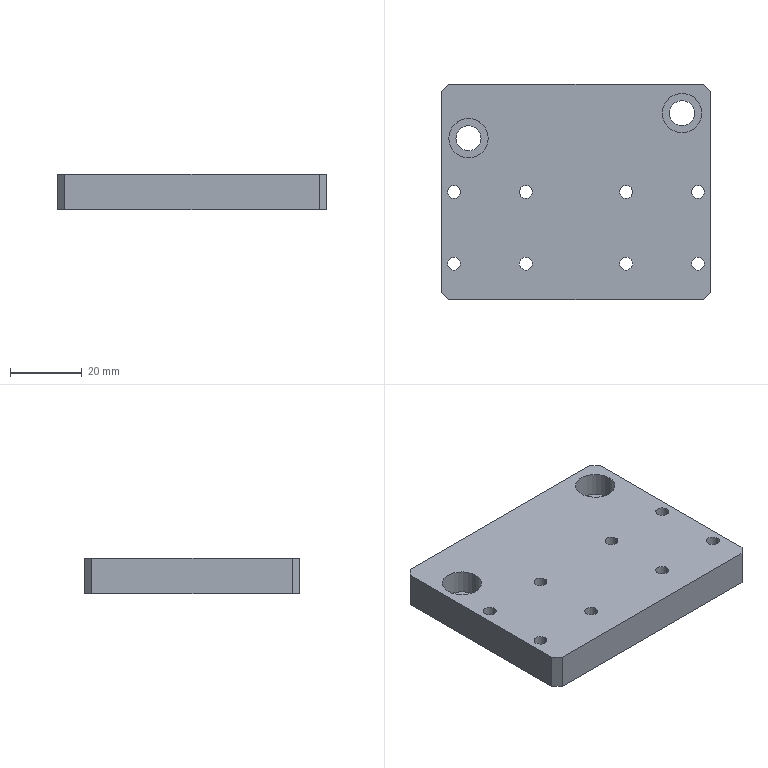Component | SolidWorks | 8TC-A17001-90-03PressureRollerMountingPlate2-1 | 1 solid | 64 faces | box 75 x 60 x 10 mm | volume 41711 mm3 | cylinder 42 | plane 20 | cone 2 | commonest cylinder face diameters 6 x16 3.6 x16 11 x4 7 x4 5 x2 | material A3
build123d program:
from build123d import *

# Parameters (mm, degrees)
SKETCH1_W                                         = 75
SKETCH1_H                                         = 60
BOSS_EXTRUDE1_DEPTH                               = 10
HOLE_SIZE_ACCORDING_TO_HEXAGON_SOCKET_D           = 3.6
HOLE_SIZE_ACCORDING_TO_HEXAGON_SOCKET_CBORE_D     = 6
HOLE_SIZE_ACCORDING_TO_HEXAGON_SOCKET_CBORE_DEPTH = 3.4
HOLE_SIZE_ACCORDING_TO_HEXAGON_SO_2_D             = 7
HOLE_SIZE_ACCORDING_TO_HEXAGON_SO_2_CBORE_D       = 11
HOLE_SIZE_ACCORDING_TO_HEXAGON_SO_2_CBORE_DEPTH   = 6.8
CHAMFER1_SIZE                                     = 2
M6_TAPPED_HOLE1_D                                 = 5
M6_TAPPED_HOLE1_DEPTH                             = 18
M6_TAPPED_HOLE1_TIP                               = 1.502


with BuildPart() as part:
    # Sketch1 → Boss-Extrude1 (new body)
    with BuildSketch(Plane.XY):
        Rectangle(SKETCH1_W, SKETCH1_H)
    extrude(amount=BOSS_EXTRUDE1_DEPTH)

    # Hole Size _ according to_ Hexagon Socket (through all)
    with Locations(Plane.XY.offset(10)):
        with Locations((-34, 20), (-34, 0), (-14, 20), (-14, 0), (14, 20), (34, 20), (14, 0), (34, 0)):
            CounterBoreHole(HOLE_SIZE_ACCORDING_TO_HEXAGON_SOCKET_D / 2, HOLE_SIZE_ACCORDING_TO_HEXAGON_SOCKET_CBORE_D / 2, HOLE_SIZE_ACCORDING_TO_HEXAGON_SOCKET_CBORE_DEPTH)

    # Hole Size _ according to_ Hexagon So 2 (through all)
    with Locations(Plane(origin=(0, 0, 0), x_dir=(-1, 0, 0), z_dir=(0, 0, -1))):
        with Locations((30, -15), (-29.59, -22)):
            CounterBoreHole(HOLE_SIZE_ACCORDING_TO_HEXAGON_SO_2_D / 2, HOLE_SIZE_ACCORDING_TO_HEXAGON_SO_2_CBORE_D / 2, HOLE_SIZE_ACCORDING_TO_HEXAGON_SO_2_CBORE_DEPTH)

    # Chamfer1
    chamfer1_edges = [part.edges().sort_by_distance(p)[0] for p in [
        (-37.5, 30, 5),
        (37.5, 30, 5),
        (37.5, -30, 5),
        (-37.5, -30, 5),
    ]]
    chamfer(chamfer1_edges, length=CHAMFER1_SIZE)

    # M6 Tapped Hole1
    with Locations(Plane(origin=(0, -30, 0), x_dir=(-1, 0, 0), z_dir=(0, -1, 0))):
        with Locations((9, -5)):
            Hole(M6_TAPPED_HOLE1_D / 2, depth=M6_TAPPED_HOLE1_DEPTH)
            with Locations((0, 0, -(M6_TAPPED_HOLE1_DEPTH + M6_TAPPED_HOLE1_TIP / 2))):  # 118° drill point
                Cone(0, M6_TAPPED_HOLE1_D / 2, M6_TAPPED_HOLE1_TIP, mode=Mode.SUBTRACT)


solid = part.part

# Placed as in the assembly
solid = solid.moved(Location((0, 23.724, -13), (180, 0, 0)))